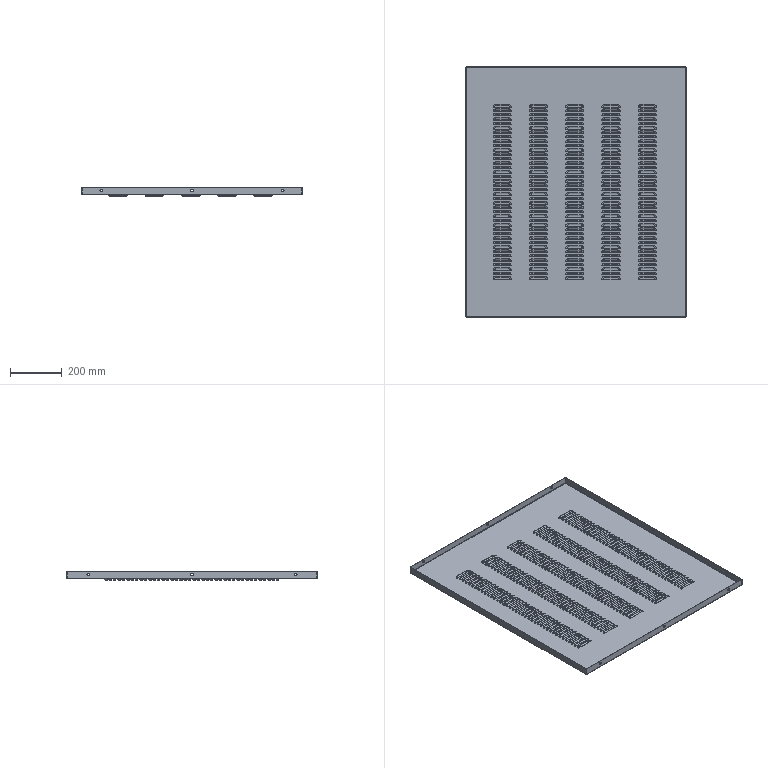Component | SolidWorks | 39RearCoverI-2 | 1 solid | 2062 faces | volume 1902193 mm3 | plane 822 | torus 800 | cylinder 432 | spline 8 | commonest cylinder face diameters 10 x224 14 x200 2 x4 6 x4